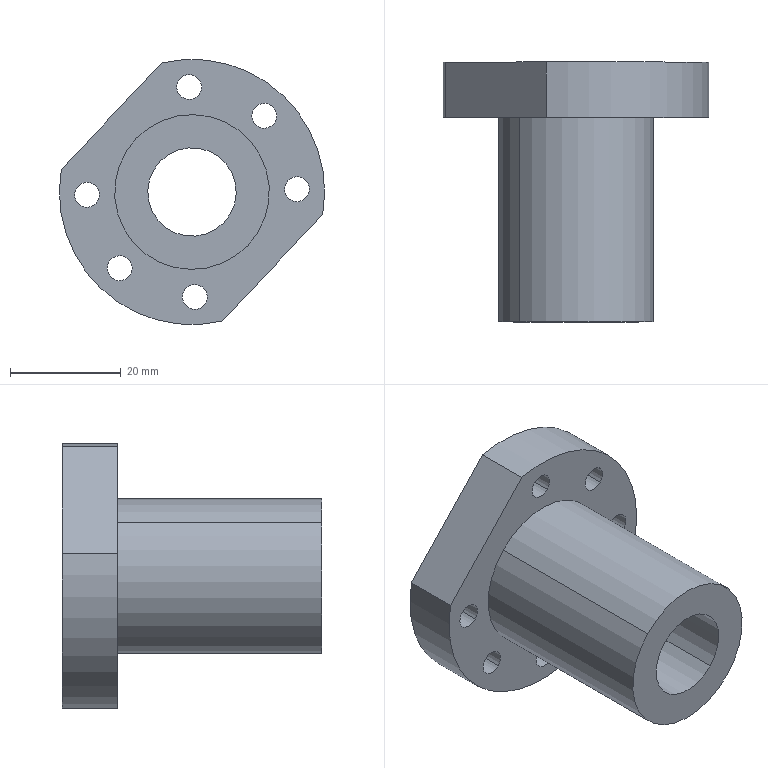Component | SolidWorks | 100-1_Copy(2)-1 | 1 solid | 23 faces | box 48 x 47 x 48 mm | volume 29034 mm3 | cylinder 18 | plane 5 | commonest cylinder face diameters 4.5 x12 16 x2 28 x2 48 x2
STEP:
#1=COLOUR_RGB('',0.7922,0.8196,0.9333);
#2=FILL_AREA_STYLE_COLOUR('',#1);
#3=FILL_AREA_STYLE('',(#2));
#4=SURFACE_STYLE_FILL_AREA(#3);
#5=SURFACE_SIDE_STYLE('',(#4));
#6=SURFACE_STYLE_USAGE(.BOTH.,#5);
#7=PRESENTATION_STYLE_ASSIGNMENT((#6));
#8=CARTESIAN_POINT('',(19.805,43.68,-79.282));
#9=VERTEX_POINT('',#8);
#10=CARTESIAN_POINT('',(19.805,45.53,-79.282));
#11=VERTEX_POINT('',#10);
#12=CARTESIAN_POINT('',(19.805,43.68,-79.282));
#13=DIRECTION('',(-0.,1.,0.));
#14=VECTOR('',#13,39.37);
#15=LINE('',#12,#14);
#16=EDGE_CURVE('',#9,#11,#15,.T.);
#17=ORIENTED_EDGE('',*,*,#16,.F.);
#18=CARTESIAN_POINT('',(19.348,43.68,-78.848));
#19=VERTEX_POINT('',#18);
#20=CARTESIAN_POINT('',(19.576,43.68,-79.065));
#21=DIRECTION('',(-0.,1.,0.));
#22=DIRECTION('',(-0.7258,0.,0.6879));
#23=AXIS2_PLACEMENT_3D('',#20,#21,#22);
#24=CIRCLE('',#23,0.315);
#25=EDGE_CURVE('',#19,#9,#24,.T.);
#26=ORIENTED_EDGE('',*,*,#25,.F.);
#27=CARTESIAN_POINT('',(19.348,45.53,-78.848));
#28=VERTEX_POINT('',#27);
#29=CARTESIAN_POINT('',(19.348,43.68,-78.848));
#30=DIRECTION('',(-0.,1.,0.));
#31=VECTOR('',#30,39.37);
#32=LINE('',#29,#31);
#33=EDGE_CURVE('',#19,#28,#32,.T.);
#34=ORIENTED_EDGE('',*,*,#33,.T.);
#35=CARTESIAN_POINT('',(19.576,45.53,-79.065));
#36=DIRECTION('',(-0.,1.,0.));
#37=DIRECTION('',(-0.7258,0.,0.6879));
#38=AXIS2_PLACEMENT_3D('',#35,#36,#37);
#39=CIRCLE('',#38,0.315);
#40=EDGE_CURVE('',#28,#11,#39,.T.);
#41=ORIENTED_EDGE('',*,*,#40,.T.);
#42=EDGE_LOOP('',(#17,#26,#34,#41));
#43=FACE_OUTER_BOUND('',#42,.T.);
#44=CARTESIAN_POINT('',(19.576,43.68,-79.065));
#45=DIRECTION('',(-0.,1.,0.));
#46=DIRECTION('',(-0.7258,0.,0.6879));
#47=AXIS2_PLACEMENT_3D('',#44,#45,#46);
#48=CYLINDRICAL_SURFACE('',#47,0.315);
#49=ADVANCED_FACE('',(#43),#48,.F.);
#50=ORIENTED_EDGE('',*,*,#25,.T.);
#51=CARTESIAN_POINT('',(19.576,43.68,-79.065));
#52=DIRECTION('',(-0.,1.,0.));
#53=DIRECTION('',(-0.7258,0.,0.6879));
#54=AXIS2_PLACEMENT_3D('',#51,#52,#53);
#55=CIRCLE('',#54,0.315);
#56=EDGE_CURVE('',#9,#19,#55,.T.);
#57=ORIENTED_EDGE('',*,*,#56,.T.);
#58=EDGE_LOOP('',(#50,#57));
#59=FACE_BOUND('',#58,.T.);
#60=CARTESIAN_POINT('',(19.176,43.68,-78.686));
#61=VERTEX_POINT('',#60);
#62=CARTESIAN_POINT('',(19.976,43.68,-79.444));
#63=VERTEX_POINT('',#62);
#64=CARTESIAN_POINT('',(19.576,43.68,-79.065));
#65=DIRECTION('',(0.,-1.,-0.));
#66=DIRECTION('',(0.7258,0.,-0.6879));
#67=AXIS2_PLACEMENT_3D('',#64,#65,#66);
#68=CIRCLE('',#67,0.5512);
#69=EDGE_CURVE('',#61,#63,#68,.T.);
#70=ORIENTED_EDGE('',*,*,#69,.T.);
#71=CARTESIAN_POINT('',(19.576,43.68,-79.065));
#72=DIRECTION('',(0.,-1.,-0.));
#73=DIRECTION('',(0.7258,0.,-0.6879));
#74=AXIS2_PLACEMENT_3D('',#71,#72,#73);
#75=CIRCLE('',#74,0.5512);
#76=EDGE_CURVE('',#63,#61,#75,.T.);
#77=ORIENTED_EDGE('',*,*,#76,.T.);
#78=EDGE_LOOP('',(#70,#77));
#79=FACE_OUTER_BOUND('',#78,.T.);
#80=CARTESIAN_POINT('',(19.576,43.68,-79.065));
#81=DIRECTION('',(0.,-1.,-0.));
#82=DIRECTION('',(0.7258,0.,-0.6879));
#83=AXIS2_PLACEMENT_3D('',#80,#81,#82);
#84=PLANE('',#83);
#85=ADVANCED_FACE('',(#59,#79),#84,.T.);
#86=CARTESIAN_POINT('',(19.976,45.136,-79.444));
#87=VERTEX_POINT('',#86);
#88=CARTESIAN_POINT('',(19.976,43.68,-79.444));
#89=DIRECTION('',(-0.,1.,0.));
#90=VECTOR('',#89,39.37);
#91=LINE('',#88,#90);
#92=EDGE_CURVE('',#63,#87,#91,.T.);
#93=ORIENTED_EDGE('',*,*,#92,.F.);
#94=ORIENTED_EDGE('',*,*,#69,.F.);
#95=CARTESIAN_POINT('',(19.176,45.136,-78.686));
#96=VERTEX_POINT('',#95);
#97=CARTESIAN_POINT('',(19.176,43.68,-78.686));
#98=DIRECTION('',(-0.,1.,0.));
#99=VECTOR('',#98,39.37);
#100=LINE('',#97,#99);
#101=EDGE_CURVE('',#61,#96,#100,.T.);
#102=ORIENTED_EDGE('',*,*,#101,.T.);
#103=CARTESIAN_POINT('',(19.576,45.136,-79.065));
#104=DIRECTION('',(0.,-1.,-0.));
#105=DIRECTION('',(-0.7258,0.,0.6879));
#106=AXIS2_PLACEMENT_3D('',#103,#104,#105);
#107=CIRCLE('',#106,0.5512);
#108=EDGE_CURVE('',#96,#87,#107,.T.);
#109=ORIENTED_EDGE('',*,*,#108,.T.);
#110=EDGE_LOOP('',(#93,#94,#102,#109));
#111=FACE_OUTER_BOUND('',#110,.T.);
#112=CARTESIAN_POINT('',(19.576,43.68,-79.065));
#113=DIRECTION('',(-0.,1.,0.));
#114=DIRECTION('',(-0.7258,0.,0.6879));
#115=AXIS2_PLACEMENT_3D('',#112,#113,#114);
#116=CYLINDRICAL_SURFACE('',#115,0.5512);
#117=ADVANCED_FACE('',(#111),#116,.T.);
#118=CARTESIAN_POINT('',(20.026,45.53,-78.461));
#119=VERTEX_POINT('',#118);
#120=CARTESIAN_POINT('',(20.026,45.136,-78.461));
#121=VERTEX_POINT('',#120);
#122=CARTESIAN_POINT('',(20.026,45.136,-78.461));
#123=DIRECTION('',(0.,-1.,-0.));
#124=VECTOR('',#123,39.37);
#125=LINE('',#122,#124);
#126=EDGE_CURVE('',#119,#121,#125,.T.);
#127=ORIENTED_EDGE('',*,*,#126,.F.);
#128=CARTESIAN_POINT('',(20.155,45.53,-78.583));
#129=VERTEX_POINT('',#128);
#130=CARTESIAN_POINT('',(20.091,45.53,-78.522));
#131=DIRECTION('',(0.,-1.,-0.));
#132=DIRECTION('',(0.7258,0.,-0.6879));
#133=AXIS2_PLACEMENT_3D('',#130,#131,#132);
#134=CIRCLE('',#133,0.08858);
#135=EDGE_CURVE('',#129,#119,#134,.T.);
#136=ORIENTED_EDGE('',*,*,#135,.F.);
#137=CARTESIAN_POINT('',(20.155,45.136,-78.583));
#138=VERTEX_POINT('',#137);
#139=CARTESIAN_POINT('',(20.155,45.136,-78.583));
#140=DIRECTION('',(0.,-1.,-0.));
#141=VECTOR('',#140,39.37);
#142=LINE('',#139,#141);
#143=EDGE_CURVE('',#129,#138,#142,.T.);
#144=ORIENTED_EDGE('',*,*,#143,.T.);
#145=CARTESIAN_POINT('',(20.091,45.136,-78.522));
#146=DIRECTION('',(0.,-1.,-0.));
#147=DIRECTION('',(0.7258,0.,-0.6879));
#148=AXIS2_PLACEMENT_3D('',#145,#146,#147);
#149=CIRCLE('',#148,0.08858);
#150=EDGE_CURVE('',#138,#121,#149,.T.);
#151=ORIENTED_EDGE('',*,*,#150,.T.);
#152=EDGE_LOOP('',(#127,#136,#144,#151));
#153=FACE_OUTER_BOUND('',#152,.T.);
#154=CARTESIAN_POINT('',(20.091,45.136,-78.522));
#155=DIRECTION('',(0.,-1.,-0.));
#156=DIRECTION('',(0.7258,0.,-0.6879));
#157=AXIS2_PLACEMENT_3D('',#154,#155,#156);
#158=CYLINDRICAL_SURFACE('',#157,0.08858);
#159=ADVANCED_FACE('',(#153),#158,.F.);
#160=CARTESIAN_POINT('',(19.492,45.53,-78.256));
#161=VERTEX_POINT('',#160);
#162=CARTESIAN_POINT('',(19.492,45.136,-78.256));
#163=VERTEX_POINT('',#162);
#164=CARTESIAN_POINT('',(19.492,45.136,-78.256));
#165=DIRECTION('',(0.,-1.,-0.));
#166=VECTOR('',#165,39.37);
#167=LINE('',#164,#166);
#168=EDGE_CURVE('',#161,#163,#167,.T.);
#169=ORIENTED_EDGE('',*,*,#168,.F.);
#170=CARTESIAN_POINT('',(19.62,45.53,-78.378));
#171=VERTEX_POINT('',#170);
#172=CARTESIAN_POINT('',(19.556,45.53,-78.317));
#173=DIRECTION('',(0.,-1.,-0.));
#174=DIRECTION('',(0.7258,0.,-0.6879));
#175=AXIS2_PLACEMENT_3D('',#172,#173,#174);
#176=CIRCLE('',#175,0.08858);
#177=EDGE_CURVE('',#171,#161,#176,.T.);
#178=ORIENTED_EDGE('',*,*,#177,.F.);
#179=CARTESIAN_POINT('',(19.62,45.136,-78.378));
#180=VERTEX_POINT('',#179);
#181=CARTESIAN_POINT('',(19.62,45.136,-78.378));
#182=DIRECTION('',(0.,-1.,-0.));
#183=VECTOR('',#182,39.37);
#184=LINE('',#181,#183);
#185=EDGE_CURVE('',#171,#180,#184,.T.);
#186=ORIENTED_EDGE('',*,*,#185,.T.);
#187=CARTESIAN_POINT('',(19.556,45.136,-78.317));
#188=DIRECTION('',(0.,-1.,-0.));
#189=DIRECTION('',(0.7258,0.,-0.6879));
#190=AXIS2_PLACEMENT_3D('',#187,#188,#189);
#191=CIRCLE('',#190,0.08858);
#192=EDGE_CURVE('',#180,#163,#191,.T.);
#193=ORIENTED_EDGE('',*,*,#192,.T.);
#194=EDGE_LOOP('',(#169,#178,#186,#193));
#195=FACE_OUTER_BOUND('',#194,.T.);
#196=CARTESIAN_POINT('',(19.556,45.136,-78.317));
#197=DIRECTION('',(0.,-1.,-0.));
#198=DIRECTION('',(0.7258,0.,-0.6879));
#199=AXIS2_PLACEMENT_3D('',#196,#197,#198);
#200=CYLINDRICAL_SURFACE('',#199,0.08858);
#201=ADVANCED_FACE('',(#195),#200,.F.);
#202=CARTESIAN_POINT('',(18.764,45.53,-79.024));
#203=VERTEX_POINT('',#202);
#204=CARTESIAN_POINT('',(18.764,45.136,-79.024));
#205=VERTEX_POINT('',#204);
#206=CARTESIAN_POINT('',(18.764,45.136,-79.024));
#207=DIRECTION('',(0.,-1.,-0.));
#208=VECTOR('',#207,39.37);
#209=LINE('',#206,#208);
#210=EDGE_CURVE('',#203,#205,#209,.T.);
#211=ORIENTED_EDGE('',*,*,#210,.F.);
#212=CARTESIAN_POINT('',(18.893,45.53,-79.146));
#213=VERTEX_POINT('',#212);
#214=CARTESIAN_POINT('',(18.828,45.53,-79.085));
#215=DIRECTION('',(0.,-1.,-0.));
#216=DIRECTION('',(0.7258,0.,-0.6879));
#217=AXIS2_PLACEMENT_3D('',#214,#215,#216);
#218=CIRCLE('',#217,0.08858);
#219=EDGE_CURVE('',#213,#203,#218,.T.);
#220=ORIENTED_EDGE('',*,*,#219,.F.);
#221=CARTESIAN_POINT('',(18.893,45.136,-79.146));
#222=VERTEX_POINT('',#221);
#223=CARTESIAN_POINT('',(18.893,45.136,-79.146));
#224=DIRECTION('',(0.,-1.,-0.));
#225=VECTOR('',#224,39.37);
#226=LINE('',#223,#225);
#227=EDGE_CURVE('',#213,#222,#226,.T.);
#228=ORIENTED_EDGE('',*,*,#227,.T.);
#229=CARTESIAN_POINT('',(18.828,45.136,-79.085));
#230=DIRECTION('',(0.,-1.,-0.));
#231=DIRECTION('',(0.7258,0.,-0.6879));
#232=AXIS2_PLACEMENT_3D('',#229,#230,#231);
#233=CIRCLE('',#232,0.08858);
#234=EDGE_CURVE('',#222,#205,#233,.T.);
#235=ORIENTED_EDGE('',*,*,#234,.T.);
#236=EDGE_LOOP('',(#211,#220,#228,#235));
#237=FACE_OUTER_BOUND('',#236,.T.);
#238=CARTESIAN_POINT('',(18.828,45.136,-79.085));
#239=DIRECTION('',(0.,-1.,-0.));
#240=DIRECTION('',(0.7258,0.,-0.6879));
#241=AXIS2_PLACEMENT_3D('',#238,#239,#240);
#242=CYLINDRICAL_SURFACE('',#241,0.08858);
#243=ADVANCED_FACE('',(#237),#242,.F.);
#244=CARTESIAN_POINT('',(19.532,45.53,-79.752));
#245=VERTEX_POINT('',#244);
#246=CARTESIAN_POINT('',(19.532,45.136,-79.752));
#247=VERTEX_POINT('',#246);
#248=CARTESIAN_POINT('',(19.532,45.136,-79.752));
#249=DIRECTION('',(0.,-1.,-0.));
#250=VECTOR('',#249,39.37);
#251=LINE('',#248,#250);
#252=EDGE_CURVE('',#245,#247,#251,.T.);
#253=ORIENTED_EDGE('',*,*,#252,.F.);
#254=CARTESIAN_POINT('',(19.66,45.53,-79.874));
#255=VERTEX_POINT('',#254);
#256=CARTESIAN_POINT('',(19.596,45.53,-79.813));
#257=DIRECTION('',(0.,-1.,-0.));
#258=DIRECTION('',(0.7258,0.,-0.6879));
#259=AXIS2_PLACEMENT_3D('',#256,#257,#258);
#260=CIRCLE('',#259,0.08858);
#261=EDGE_CURVE('',#255,#245,#260,.T.);
#262=ORIENTED_EDGE('',*,*,#261,.F.);
#263=CARTESIAN_POINT('',(19.66,45.136,-79.874));
#264=VERTEX_POINT('',#263);
#265=CARTESIAN_POINT('',(19.66,45.136,-79.874));
#266=DIRECTION('',(0.,-1.,-0.));
#267=VECTOR('',#266,39.37);
#268=LINE('',#265,#267);
#269=EDGE_CURVE('',#255,#264,#268,.T.);
#270=ORIENTED_EDGE('',*,*,#269,.T.);
#271=CARTESIAN_POINT('',(19.596,45.136,-79.813));
#272=DIRECTION('',(0.,-1.,-0.));
#273=DIRECTION('',(0.7258,0.,-0.6879));
#274=AXIS2_PLACEMENT_3D('',#271,#272,#273);
#275=CIRCLE('',#274,0.08858);
#276=EDGE_CURVE('',#264,#247,#275,.T.);
#277=ORIENTED_EDGE('',*,*,#276,.T.);
#278=EDGE_LOOP('',(#253,#262,#270,#277));
#279=FACE_OUTER_BOUND('',#278,.T.);
#280=CARTESIAN_POINT('',(19.596,45.136,-79.813));
#281=DIRECTION('',(0.,-1.,-0.));
#282=DIRECTION('',(0.7258,0.,-0.6879));
#283=AXIS2_PLACEMENT_3D('',#280,#281,#282);
#284=CYLINDRICAL_SURFACE('',#283,0.08858);
#285=ADVANCED_FACE('',(#279),#284,.F.);
#286=CARTESIAN_POINT('',(18.997,45.53,-79.547));
#287=VERTEX_POINT('',#286);
#288=CARTESIAN_POINT('',(18.997,45.136,-79.547));
#289=VERTEX_POINT('',#288);
#290=CARTESIAN_POINT('',(18.997,45.136,-79.547));
#291=DIRECTION('',(0.,-1.,-0.));
#292=VECTOR('',#291,39.37);
#293=LINE('',#290,#292);
#294=EDGE_CURVE('',#287,#289,#293,.T.);
#295=ORIENTED_EDGE('',*,*,#294,.F.);
#296=CARTESIAN_POINT('',(19.126,45.53,-79.669));
#297=VERTEX_POINT('',#296);
#298=CARTESIAN_POINT('',(19.062,45.53,-79.608));
#299=DIRECTION('',(0.,-1.,-0.));
#300=DIRECTION('',(0.7258,0.,-0.6879));
#301=AXIS2_PLACEMENT_3D('',#298,#299,#300);
#302=CIRCLE('',#301,0.08858);
#303=EDGE_CURVE('',#297,#287,#302,.T.);
#304=ORIENTED_EDGE('',*,*,#303,.F.);
#305=CARTESIAN_POINT('',(19.126,45.136,-79.669));
#306=VERTEX_POINT('',#305);
#307=CARTESIAN_POINT('',(19.126,45.136,-79.669));
#308=DIRECTION('',(0.,-1.,-0.));
#309=VECTOR('',#308,39.37);
#310=LINE('',#307,#309);
#311=EDGE_CURVE('',#297,#306,#310,.T.);
#312=ORIENTED_EDGE('',*,*,#311,.T.);
#313=CARTESIAN_POINT('',(19.062,45.136,-79.608));
#314=DIRECTION('',(0.,-1.,-0.));
#315=DIRECTION('',(0.7258,0.,-0.6879));
#316=AXIS2_PLACEMENT_3D('',#313,#314,#315);
#317=CIRCLE('',#316,0.08858);
#318=EDGE_CURVE('',#306,#289,#317,.T.);
#319=ORIENTED_EDGE('',*,*,#318,.T.);
#320=EDGE_LOOP('',(#295,#304,#312,#319));
#321=FACE_OUTER_BOUND('',#320,.T.);
#322=CARTESIAN_POINT('',(19.062,45.136,-79.608));
#323=DIRECTION('',(0.,-1.,-0.));
#324=DIRECTION('',(0.7258,0.,-0.6879));
#325=AXIS2_PLACEMENT_3D('',#322,#323,#324);
#326=CYLINDRICAL_SURFACE('',#325,0.08858);
#327=ADVANCED_FACE('',(#321),#326,.F.);
#328=CARTESIAN_POINT('',(20.26,45.53,-78.984));
#329=VERTEX_POINT('',#328);
#330=CARTESIAN_POINT('',(20.26,45.136,-78.984));
#331=VERTEX_POINT('',#330);
#332=CARTESIAN_POINT('',(20.26,45.136,-78.984));
#333=DIRECTION('',(0.,-1.,-0.));
#334=VECTOR('',#333,39.37);
#335=LINE('',#332,#334);
#336=EDGE_CURVE('',#329,#331,#335,.T.);
#337=ORIENTED_EDGE('',*,*,#336,.F.);
#338=CARTESIAN_POINT('',(20.388,45.53,-79.106));
#339=VERTEX_POINT('',#338);
#340=CARTESIAN_POINT('',(20.324,45.53,-79.045));
#341=DIRECTION('',(0.,-1.,-0.));
#342=DIRECTION('',(0.7258,0.,-0.6879));
#343=AXIS2_PLACEMENT_3D('',#340,#341,#342);
#344=CIRCLE('',#343,0.08858);
#345=EDGE_CURVE('',#339,#329,#344,.T.);
#346=ORIENTED_EDGE('',*,*,#345,.F.);
#347=CARTESIAN_POINT('',(20.388,45.136,-79.106));
#348=VERTEX_POINT('',#347);
#349=CARTESIAN_POINT('',(20.388,45.136,-79.106));
#350=DIRECTION('',(0.,-1.,-0.));
#351=VECTOR('',#350,39.37);
#352=LINE('',#349,#351);
#353=EDGE_CURVE('',#339,#348,#352,.T.);
#354=ORIENTED_EDGE('',*,*,#353,.T.);
#355=CARTESIAN_POINT('',(20.324,45.136,-79.045));
#356=DIRECTION('',(0.,-1.,-0.));
#357=DIRECTION('',(0.7258,0.,-0.6879));
#358=AXIS2_PLACEMENT_3D('',#355,#356,#357);
#359=CIRCLE('',#358,0.08858);
#360=EDGE_CURVE('',#348,#331,#359,.T.);
#361=ORIENTED_EDGE('',*,*,#360,.T.);
#362=EDGE_LOOP('',(#337,#346,#354,#361));
#363=FACE_OUTER_BOUND('',#362,.T.);
#364=CARTESIAN_POINT('',(20.324,45.136,-79.045));
#365=DIRECTION('',(0.,-1.,-0.));
#366=DIRECTION('',(0.7258,0.,-0.6879));
#367=AXIS2_PLACEMENT_3D('',#364,#365,#366);
#368=CYLINDRICAL_SURFACE('',#367,0.08858);
#369=ADVANCED_FACE('',(#363),#368,.F.);
#370=ORIENTED_EDGE('',*,*,#345,.T.);
#371=CARTESIAN_POINT('',(20.324,45.53,-79.045));
#372=DIRECTION('',(0.,-1.,-0.));
#373=DIRECTION('',(0.7258,0.,-0.6879));
#374=AXIS2_PLACEMENT_3D('',#371,#372,#373);
#375=CIRCLE('',#374,0.08858);
#376=EDGE_CURVE('',#329,#339,#375,.T.);
#377=ORIENTED_EDGE('',*,*,#376,.T.);
#378=EDGE_LOOP('',(#370,#377));
#379=FACE_BOUND('',#378,.T.);
#380=ORIENTED_EDGE('',*,*,#303,.T.);
#381=CARTESIAN_POINT('',(19.062,45.53,-79.608));
#382=DIRECTION('',(0.,-1.,-0.));
#383=DIRECTION('',(0.7258,0.,-0.6879));
#384=AXIS2_PLACEMENT_3D('',#381,#382,#383);
#385=CIRCLE('',#384,0.08858);
#386=EDGE_CURVE('',#287,#297,#385,.T.);
#387=ORIENTED_EDGE('',*,*,#386,.T.);
#388=EDGE_LOOP('',(#380,#387));
#389=FACE_BOUND('',#388,.T.);
#390=ORIENTED_EDGE('',*,*,#261,.T.);
#391=CARTESIAN_POINT('',(19.596,45.53,-79.813));
#392=DIRECTION('',(0.,-1.,-0.));
#393=DIRECTION('',(0.7258,0.,-0.6879));
#394=AXIS2_PLACEMENT_3D('',#391,#392,#393);
#395=CIRCLE('',#394,0.08858);
#396=EDGE_CURVE('',#245,#255,#395,.T.);
#397=ORIENTED_EDGE('',*,*,#396,.T.);
#398=EDGE_LOOP('',(#390,#397));
#399=FACE_BOUND('',#398,.T.);
#400=ORIENTED_EDGE('',*,*,#219,.T.);
#401=CARTESIAN_POINT('',(18.828,45.53,-79.085));
#402=DIRECTION('',(0.,-1.,-0.));
#403=DIRECTION('',(0.7258,0.,-0.6879));
#404=AXIS2_PLACEMENT_3D('',#401,#402,#403);
#405=CIRCLE('',#404,0.08858);
#406=EDGE_CURVE('',#203,#213,#405,.T.);
#407=ORIENTED_EDGE('',*,*,#406,.T.);
#408=EDGE_LOOP('',(#400,#407));
#409=FACE_BOUND('',#408,.T.);
#410=ORIENTED_EDGE('',*,*,#177,.T.);
#411=CARTESIAN_POINT('',(19.556,45.53,-78.317));
#412=DIRECTION('',(0.,-1.,-0.));
#413=DIRECTION('',(0.7258,0.,-0.6879));
#414=AXIS2_PLACEMENT_3D('',#411,#412,#413);
#415=CIRCLE('',#414,0.08858);
#416=EDGE_CURVE('',#161,#171,#415,.T.);
#417=ORIENTED_EDGE('',*,*,#416,.T.);
#418=EDGE_LOOP('',(#410,#417));
#419=FACE_BOUND('',#418,.T.);
#420=ORIENTED_EDGE('',*,*,#135,.T.);
#421=CARTESIAN_POINT('',(20.091,45.53,-78.522));
#422=DIRECTION('',(0.,-1.,-0.));
#423=DIRECTION('',(0.7258,0.,-0.6879));
#424=AXIS2_PLACEMENT_3D('',#421,#422,#423);
#425=CIRCLE('',#424,0.08858);
#426=EDGE_CURVE('',#119,#129,#425,.T.);
#427=ORIENTED_EDGE('',*,*,#426,.T.);
#428=EDGE_LOOP('',(#420,#427));
#429=FACE_BOUND('',#428,.T.);
#430=ORIENTED_EDGE('',*,*,#40,.F.);
#431=CARTESIAN_POINT('',(19.576,45.53,-79.065));
#432=DIRECTION('',(-0.,1.,0.));
#433=DIRECTION('',(-0.7258,0.,0.6879));
#434=AXIS2_PLACEMENT_3D('',#431,#432,#433);
#435=CIRCLE('',#434,0.315);
#436=EDGE_CURVE('',#11,#28,#435,.T.);
#437=ORIENTED_EDGE('',*,*,#436,.F.);
#438=EDGE_LOOP('',(#430,#437));
#439=FACE_BOUND('',#438,.T.);
#440=CARTESIAN_POINT('',(19.364,45.53,-78.144));
#441=VERTEX_POINT('',#440);
#442=CARTESIAN_POINT('',(20.507,45.53,-79.227));
#443=VERTEX_POINT('',#442);
#444=CARTESIAN_POINT('',(19.576,45.53,-79.065));
#445=DIRECTION('',(-0.,1.,0.));
#446=DIRECTION('',(-0.7258,0.,0.6879));
#447=AXIS2_PLACEMENT_3D('',#444,#445,#446);
#448=CIRCLE('',#447,0.9449);
#449=EDGE_CURVE('',#441,#443,#448,.T.);
#450=ORIENTED_EDGE('',*,*,#449,.T.);
#451=CARTESIAN_POINT('',(19.788,45.53,-79.986));
#452=VERTEX_POINT('',#451);
#453=CARTESIAN_POINT('',(20.507,45.53,-79.227));
#454=DIRECTION('',(-0.6879,-0.,-0.7258));
#455=VECTOR('',#454,39.37);
#456=LINE('',#453,#455);
#457=EDGE_CURVE('',#443,#452,#456,.T.);
#458=ORIENTED_EDGE('',*,*,#457,.T.);
#459=CARTESIAN_POINT('',(18.645,45.53,-78.902));
#460=VERTEX_POINT('',#459);
#461=CARTESIAN_POINT('',(19.576,45.53,-79.065));
#462=DIRECTION('',(-0.,1.,0.));
#463=DIRECTION('',(-0.7258,0.,0.6879));
#464=AXIS2_PLACEMENT_3D('',#461,#462,#463);
#465=CIRCLE('',#464,0.9449);
#466=EDGE_CURVE('',#452,#460,#465,.T.);
#467=ORIENTED_EDGE('',*,*,#466,.T.);
#468=CARTESIAN_POINT('',(18.645,45.53,-78.902));
#469=DIRECTION('',(0.6879,0.,0.7258));
#470=VECTOR('',#469,39.37);
#471=LINE('',#468,#470);
#472=EDGE_CURVE('',#460,#441,#471,.T.);
#473=ORIENTED_EDGE('',*,*,#472,.T.);
#474=EDGE_LOOP('',(#450,#458,#467,#473));
#475=FACE_OUTER_BOUND('',#474,.T.);
#476=CARTESIAN_POINT('',(19.576,45.53,-79.065));
#477=DIRECTION('',(-0.,1.,0.));
#478=DIRECTION('',(0.6879,0.,0.7258));
#479=AXIS2_PLACEMENT_3D('',#476,#477,#478);
#480=PLANE('',#479);
#481=ADVANCED_FACE('',(#379,#389,#399,#409,#419,#429,#439,#475),#480,.T.);
#482=CARTESIAN_POINT('',(18.645,45.136,-78.902));
#483=VERTEX_POINT('',#482);
#484=CARTESIAN_POINT('',(19.364,45.136,-78.144));
#485=VERTEX_POINT('',#484);
#486=CARTESIAN_POINT('',(18.645,45.136,-78.902));
#487=DIRECTION('',(0.6879,0.,0.7258));
#488=VECTOR('',#487,39.37);
#489=LINE('',#486,#488);
#490=EDGE_CURVE('',#483,#485,#489,.T.);
#491=ORIENTED_EDGE('',*,*,#490,.T.);
#492=CARTESIAN_POINT('',(19.364,45.53,-78.144));
#493=DIRECTION('',(0.,-1.,-0.));
#494=VECTOR('',#493,39.37);
#495=LINE('',#492,#494);
#496=EDGE_CURVE('',#441,#485,#495,.T.);
#497=ORIENTED_EDGE('',*,*,#496,.F.);
#498=ORIENTED_EDGE('',*,*,#472,.F.);
#499=CARTESIAN_POINT('',(18.645,45.53,-78.902));
#500=DIRECTION('',(0.,-1.,-0.));
#501=VECTOR('',#500,39.37);
#502=LINE('',#499,#501);
#503=EDGE_CURVE('',#460,#483,#502,.T.);
#504=ORIENTED_EDGE('',*,*,#503,.T.);
#505=EDGE_LOOP('',(#491,#497,#498,#504));
#506=FACE_OUTER_BOUND('',#505,.T.);
#507=CARTESIAN_POINT('',(18.645,45.53,-78.902));
#508=DIRECTION('',(0.7258,0.,-0.6879));
#509=DIRECTION('',(-0.6879,-0.,-0.7258));
#510=AXIS2_PLACEMENT_3D('',#507,#508,#509);
#511=PLANE('',#510);
#512=ADVANCED_FACE('',(#506),#511,.F.);
#513=CARTESIAN_POINT('',(19.788,45.136,-79.986));
#514=VERTEX_POINT('',#513);
#515=CARTESIAN_POINT('',(19.576,45.136,-79.065));
#516=DIRECTION('',(-0.,1.,0.));
#517=DIRECTION('',(-0.7258,0.,0.6879));
#518=AXIS2_PLACEMENT_3D('',#515,#516,#517);
#519=CIRCLE('',#518,0.9449);
#520=EDGE_CURVE('',#514,#483,#519,.T.);
#521=ORIENTED_EDGE('',*,*,#520,.T.);
#522=ORIENTED_EDGE('',*,*,#503,.F.);
#523=ORIENTED_EDGE('',*,*,#466,.F.);
#524=CARTESIAN_POINT('',(19.788,45.53,-79.986));
#525=DIRECTION('',(0.,-1.,-0.));
#526=VECTOR('',#525,39.37);
#527=LINE('',#524,#526);
#528=EDGE_CURVE('',#452,#514,#527,.T.);
#529=ORIENTED_EDGE('',*,*,#528,.T.);
#530=EDGE_LOOP('',(#521,#522,#523,#529));
#531=FACE_OUTER_BOUND('',#530,.T.);
#532=CARTESIAN_POINT('',(19.576,45.53,-79.065));
#533=DIRECTION('',(0.,-1.,-0.));
#534=DIRECTION('',(0.7258,0.,-0.6879));
#535=AXIS2_PLACEMENT_3D('',#532,#533,#534);
#536=CYLINDRICAL_SURFACE('',#535,0.9449);
#537=ADVANCED_FACE('',(#531),#536,.T.);
#538=CARTESIAN_POINT('',(20.507,45.136,-79.227));
#539=VERTEX_POINT('',#538);
#540=CARTESIAN_POINT('',(20.507,45.136,-79.227));
#541=DIRECTION('',(-0.6879,-0.,-0.7258));
#542=VECTOR('',#541,39.37);
#543=LINE('',#540,#542);
#544=EDGE_CURVE('',#539,#514,#543,.T.);
#545=ORIENTED_EDGE('',*,*,#544,.T.);
#546=ORIENTED_EDGE('',*,*,#528,.F.);
#547=ORIENTED_EDGE('',*,*,#457,.F.);
#548=CARTESIAN_POINT('',(20.507,45.53,-79.227));
#549=DIRECTION('',(0.,-1.,-0.));
#550=VECTOR('',#549,39.37);
#551=LINE('',#548,#550);
#552=EDGE_CURVE('',#443,#539,#551,.T.);
#553=ORIENTED_EDGE('',*,*,#552,.T.);
#554=EDGE_LOOP('',(#545,#546,#547,#553));
#555=FACE_OUTER_BOUND('',#554,.T.);
#556=CARTESIAN_POINT('',(20.507,45.53,-79.227));
#557=DIRECTION('',(-0.7258,-0.,0.6879));
#558=DIRECTION('',(0.6879,0.,0.7258));
#559=AXIS2_PLACEMENT_3D('',#556,#557,#558);
#560=PLANE('',#559);
#561=ADVANCED_FACE('',(#555),#560,.F.);
#562=CARTESIAN_POINT('',(19.576,45.136,-79.065));
#563=DIRECTION('',(-0.,1.,0.));
#564=DIRECTION('',(-0.7258,0.,0.6879));
#565=AXIS2_PLACEMENT_3D('',#562,#563,#564);
#566=CIRCLE('',#565,0.9449);
#567=EDGE_CURVE('',#485,#539,#566,.T.);
#568=ORIENTED_EDGE('',*,*,#567,.T.);
#569=ORIENTED_EDGE('',*,*,#552,.F.);
#570=ORIENTED_EDGE('',*,*,#449,.F.);
#571=ORIENTED_EDGE('',*,*,#496,.T.);
#572=EDGE_LOOP('',(#568,#569,#570,#571));
#573=FACE_OUTER_BOUND('',#572,.T.);
#574=CARTESIAN_POINT('',(19.576,45.53,-79.065));
#575=DIRECTION('',(0.,-1.,-0.));
#576=DIRECTION('',(0.7258,0.,-0.6879));
#577=AXIS2_PLACEMENT_3D('',#574,#575,#576);
#578=CYLINDRICAL_SURFACE('',#577,0.9449);
#579=ADVANCED_FACE('',(#573),#578,.T.);
#580=ORIENTED_EDGE('',*,*,#108,.F.);
#581=CARTESIAN_POINT('',(19.576,45.136,-79.065));
#582=DIRECTION('',(0.,-1.,-0.));
#583=DIRECTION('',(-0.7258,0.,0.6879));
#584=AXIS2_PLACEMENT_3D('',#581,#582,#583);
#585=CIRCLE('',#584,0.5512);
#586=EDGE_CURVE('',#87,#96,#585,.T.);
#587=ORIENTED_EDGE('',*,*,#586,.F.);
#588=EDGE_LOOP('',(#580,#587));
#589=FACE_BOUND('',#588,.T.);
#590=ORIENTED_EDGE('',*,*,#360,.F.);
#591=CARTESIAN_POINT('',(20.324,45.136,-79.045));
#592=DIRECTION('',(0.,-1.,-0.));
#593=DIRECTION('',(0.7258,0.,-0.6879));
#594=AXIS2_PLACEMENT_3D('',#591,#592,#593);
#595=CIRCLE('',#594,0.08858);
#596=EDGE_CURVE('',#331,#348,#595,.T.);
#597=ORIENTED_EDGE('',*,*,#596,.F.);
#598=EDGE_LOOP('',(#590,#597));
#599=FACE_BOUND('',#598,.T.);
#600=ORIENTED_EDGE('',*,*,#318,.F.);
#601=CARTESIAN_POINT('',(19.062,45.136,-79.608));
#602=DIRECTION('',(0.,-1.,-0.));
#603=DIRECTION('',(0.7258,0.,-0.6879));
#604=AXIS2_PLACEMENT_3D('',#601,#602,#603);
#605=CIRCLE('',#604,0.08858);
#606=EDGE_CURVE('',#289,#306,#605,.T.);
#607=ORIENTED_EDGE('',*,*,#606,.F.);
#608=EDGE_LOOP('',(#600,#607));
#609=FACE_BOUND('',#608,.T.);
#610=ORIENTED_EDGE('',*,*,#276,.F.);
#611=CARTESIAN_POINT('',(19.596,45.136,-79.813));
#612=DIRECTION('',(0.,-1.,-0.));
#613=DIRECTION('',(0.7258,0.,-0.6879));
#614=AXIS2_PLACEMENT_3D('',#611,#612,#613);
#615=CIRCLE('',#614,0.08858);
#616=EDGE_CURVE('',#247,#264,#615,.T.);
#617=ORIENTED_EDGE('',*,*,#616,.F.);
#618=EDGE_LOOP('',(#610,#617));
#619=FACE_BOUND('',#618,.T.);
#620=ORIENTED_EDGE('',*,*,#234,.F.);
#621=CARTESIAN_POINT('',(18.828,45.136,-79.085));
#622=DIRECTION('',(0.,-1.,-0.));
#623=DIRECTION('',(0.7258,0.,-0.6879));
#624=AXIS2_PLACEMENT_3D('',#621,#622,#623);
#625=CIRCLE('',#624,0.08858);
#626=EDGE_CURVE('',#205,#222,#625,.T.);
#627=ORIENTED_EDGE('',*,*,#626,.F.);
#628=EDGE_LOOP('',(#620,#627));
#629=FACE_BOUND('',#628,.T.);
#630=ORIENTED_EDGE('',*,*,#192,.F.);
#631=CARTESIAN_POINT('',(19.556,45.136,-78.317));
#632=DIRECTION('',(0.,-1.,-0.));
#633=DIRECTION('',(0.7258,0.,-0.6879));
#634=AXIS2_PLACEMENT_3D('',#631,#632,#633);
#635=CIRCLE('',#634,0.08858);
#636=EDGE_CURVE('',#163,#180,#635,.T.);
#637=ORIENTED_EDGE('',*,*,#636,.F.);
#638=EDGE_LOOP('',(#630,#637));
#639=FACE_BOUND('',#638,.T.);
#640=ORIENTED_EDGE('',*,*,#150,.F.);
#641=CARTESIAN_POINT('',(20.091,45.136,-78.522));
#642=DIRECTION('',(0.,-1.,-0.));
#643=DIRECTION('',(0.7258,0.,-0.6879));
#644=AXIS2_PLACEMENT_3D('',#641,#642,#643);
#645=CIRCLE('',#644,0.08858);
#646=EDGE_CURVE('',#121,#138,#645,.T.);
#647=ORIENTED_EDGE('',*,*,#646,.F.);
#648=EDGE_LOOP('',(#640,#647));
#649=FACE_BOUND('',#648,.T.);
#650=ORIENTED_EDGE('',*,*,#567,.F.);
#651=ORIENTED_EDGE('',*,*,#490,.F.);
#652=ORIENTED_EDGE('',*,*,#520,.F.);
#653=ORIENTED_EDGE('',*,*,#544,.F.);
#654=EDGE_LOOP('',(#650,#651,#652,#653));
#655=FACE_OUTER_BOUND('',#654,.T.);
#656=CARTESIAN_POINT('',(19.576,45.136,-79.065));
#657=DIRECTION('',(-0.,1.,0.));
#658=DIRECTION('',(0.6879,0.,0.7258));
#659=AXIS2_PLACEMENT_3D('',#656,#657,#658);
#660=PLANE('',#659);
#661=ADVANCED_FACE('',(#589,#599,#609,#619,#629,#639,#649,#655),#660,.F.);
#662=ORIENTED_EDGE('',*,*,#376,.F.);
#663=ORIENTED_EDGE('',*,*,#336,.T.);
#664=ORIENTED_EDGE('',*,*,#596,.T.);
#665=ORIENTED_EDGE('',*,*,#353,.F.);
#666=EDGE_LOOP('',(#662,#663,#664,#665));
#667=FACE_OUTER_BOUND('',#666,.T.);
#668=CARTESIAN_POINT('',(20.324,45.136,-79.045));
#669=DIRECTION('',(0.,-1.,-0.));
#670=DIRECTION('',(0.7258,0.,-0.6879));
#671=AXIS2_PLACEMENT_3D('',#668,#669,#670);
#672=CYLINDRICAL_SURFACE('',#671,0.08858);
#673=ADVANCED_FACE('',(#667),#672,.F.);
#674=ORIENTED_EDGE('',*,*,#386,.F.);
#675=ORIENTED_EDGE('',*,*,#294,.T.);
#676=ORIENTED_EDGE('',*,*,#606,.T.);
#677=ORIENTED_EDGE('',*,*,#311,.F.);
#678=EDGE_LOOP('',(#674,#675,#676,#677));
#679=FACE_OUTER_BOUND('',#678,.T.);
#680=CARTESIAN_POINT('',(19.062,45.136,-79.608));
#681=DIRECTION('',(0.,-1.,-0.));
#682=DIRECTION('',(0.7258,0.,-0.6879));
#683=AXIS2_PLACEMENT_3D('',#680,#681,#682);
#684=CYLINDRICAL_SURFACE('',#683,0.08858);
#685=ADVANCED_FACE('',(#679),#684,.F.);
#686=ORIENTED_EDGE('',*,*,#396,.F.);
#687=ORIENTED_EDGE('',*,*,#252,.T.);
#688=ORIENTED_EDGE('',*,*,#616,.T.);
#689=ORIENTED_EDGE('',*,*,#269,.F.);
#690=EDGE_LOOP('',(#686,#687,#688,#689));
#691=FACE_OUTER_BOUND('',#690,.T.);
#692=CARTESIAN_POINT('',(19.596,45.136,-79.813));
#693=DIRECTION('',(0.,-1.,-0.));
#694=DIRECTION('',(0.7258,0.,-0.6879));
#695=AXIS2_PLACEMENT_3D('',#692,#693,#694);
#696=CYLINDRICAL_SURFACE('',#695,0.08858);
#697=ADVANCED_FACE('',(#691),#696,.F.);
#698=ORIENTED_EDGE('',*,*,#406,.F.);
#699=ORIENTED_EDGE('',*,*,#210,.T.);
#700=ORIENTED_EDGE('',*,*,#626,.T.);
#701=ORIENTED_EDGE('',*,*,#227,.F.);
#702=EDGE_LOOP('',(#698,#699,#700,#701));
#703=FACE_OUTER_BOUND('',#702,.T.);
#704=CARTESIAN_POINT('',(18.828,45.136,-79.085));
#705=DIRECTION('',(0.,-1.,-0.));
#706=DIRECTION('',(0.7258,0.,-0.6879));
#707=AXIS2_PLACEMENT_3D('',#704,#705,#706);
#708=CYLINDRICAL_SURFACE('',#707,0.08858);
#709=ADVANCED_FACE('',(#703),#708,.F.);
#710=ORIENTED_EDGE('',*,*,#416,.F.);
#711=ORIENTED_EDGE('',*,*,#168,.T.);
#712=ORIENTED_EDGE('',*,*,#636,.T.);
#713=ORIENTED_EDGE('',*,*,#185,.F.);
#714=EDGE_LOOP('',(#710,#711,#712,#713));
#715=FACE_OUTER_BOUND('',#714,.T.);
#716=CARTESIAN_POINT('',(19.556,45.136,-78.317));
#717=DIRECTION('',(0.,-1.,-0.));
#718=DIRECTION('',(0.7258,0.,-0.6879));
#719=AXIS2_PLACEMENT_3D('',#716,#717,#718);
#720=CYLINDRICAL_SURFACE('',#719,0.08858);
#721=ADVANCED_FACE('',(#715),#720,.F.);
#722=ORIENTED_EDGE('',*,*,#426,.F.);
#723=ORIENTED_EDGE('',*,*,#126,.T.);
#724=ORIENTED_EDGE('',*,*,#646,.T.);
#725=ORIENTED_EDGE('',*,*,#143,.F.);
#726=EDGE_LOOP('',(#722,#723,#724,#725));
#727=FACE_OUTER_BOUND('',#726,.T.);
#728=CARTESIAN_POINT('',(20.091,45.136,-78.522));
#729=DIRECTION('',(0.,-1.,-0.));
#730=DIRECTION('',(0.7258,0.,-0.6879));
#731=AXIS2_PLACEMENT_3D('',#728,#729,#730);
#732=CYLINDRICAL_SURFACE('',#731,0.08858);
#733=ADVANCED_FACE('',(#727),#732,.F.);
#734=ORIENTED_EDGE('',*,*,#76,.F.);
#735=ORIENTED_EDGE('',*,*,#92,.T.);
#736=ORIENTED_EDGE('',*,*,#586,.T.);
#737=ORIENTED_EDGE('',*,*,#101,.F.);
#738=EDGE_LOOP('',(#734,#735,#736,#737));
#739=FACE_OUTER_BOUND('',#738,.T.);
#740=CARTESIAN_POINT('',(19.576,43.68,-79.065));
#741=DIRECTION('',(-0.,1.,0.));
#742=DIRECTION('',(-0.7258,0.,0.6879));
#743=AXIS2_PLACEMENT_3D('',#740,#741,#742);
#744=CYLINDRICAL_SURFACE('',#743,0.5512);
#745=ADVANCED_FACE('',(#739),#744,.T.);
#746=ORIENTED_EDGE('',*,*,#56,.F.);
#747=ORIENTED_EDGE('',*,*,#16,.T.);
#748=ORIENTED_EDGE('',*,*,#436,.T.);
#749=ORIENTED_EDGE('',*,*,#33,.F.);
#750=EDGE_LOOP('',(#746,#747,#748,#749));
#751=FACE_OUTER_BOUND('',#750,.T.);
#752=CARTESIAN_POINT('',(19.576,43.68,-79.065));
#753=DIRECTION('',(-0.,1.,0.));
#754=DIRECTION('',(-0.7258,0.,0.6879));
#755=AXIS2_PLACEMENT_3D('',#752,#753,#754);
#756=CYLINDRICAL_SURFACE('',#755,0.315);
#757=ADVANCED_FACE('',(#751),#756,.F.);
#758=CLOSED_SHELL('',(#49,#85,#117,#159,#201,#243,#285,#327,#369,#481,#512,#537,#561,#579,#661,#673,#685,#697,#709,#721,#733,#745,#757));
#759=MANIFOLD_SOLID_BREP('',#758);
#760=STYLED_ITEM('',(#7),#759);
#761=(LENGTH_UNIT()NAMED_UNIT(*)SI_UNIT($,.METRE.));
#762=LENGTH_MEASURE_WITH_UNIT(LENGTH_MEASURE(0.0254),#761);
#763=DIMENSIONAL_EXPONENTS(1.,0.,0.,0.,0.,0.,0.);
#764=(CONVERSION_BASED_UNIT('',#762)LENGTH_UNIT()NAMED_UNIT(#763));
#765=UNCERTAINTY_MEASURE_WITH_UNIT(LENGTH_MEASURE(0.00001),#764,'','');
#766=(NAMED_UNIT(*)PLANE_ANGLE_UNIT()SI_UNIT($,.RADIAN.));
#767=(NAMED_UNIT(*)SI_UNIT($,.STERADIAN.)SOLID_ANGLE_UNIT());
#768=(GEOMETRIC_REPRESENTATION_CONTEXT(3)GLOBAL_UNCERTAINTY_ASSIGNED_CONTEXT((#765))GLOBAL_UNIT_ASSIGNED_CONTEXT((#764,#766,#767))REPRESENTATION_CONTEXT('',''));
#769=MECHANICAL_DESIGN_GEOMETRIC_PRESENTATION_REPRESENTATION('',(#760),#768);
#770=CARTESIAN_POINT('',(0.,0.,0.));
#771=DIRECTION('',(0.,0.,1.));
#772=DIRECTION('',(1.,0.,0.));
#773=AXIS2_PLACEMENT_3D('',#770,#771,#772);
#774=(LENGTH_UNIT()NAMED_UNIT(*)SI_UNIT($,.METRE.));
#775=LENGTH_MEASURE_WITH_UNIT(LENGTH_MEASURE(0.0254),#774);
#776=DIMENSIONAL_EXPONENTS(1.,0.,0.,0.,0.,0.,0.);
#777=(CONVERSION_BASED_UNIT('',#775)LENGTH_UNIT()NAMED_UNIT(#776));
#778=UNCERTAINTY_MEASURE_WITH_UNIT(LENGTH_MEASURE(0.00001),#777,'','');
#779=(NAMED_UNIT(*)PLANE_ANGLE_UNIT()SI_UNIT($,.RADIAN.));
#780=(NAMED_UNIT(*)SI_UNIT($,.STERADIAN.)SOLID_ANGLE_UNIT());
#781=(GEOMETRIC_REPRESENTATION_CONTEXT(3)GLOBAL_UNCERTAINTY_ASSIGNED_CONTEXT((#778))GLOBAL_UNIT_ASSIGNED_CONTEXT((#777,#779,#780))REPRESENTATION_CONTEXT('',''));
#782=ADVANCED_BREP_SHAPE_REPRESENTATION('',(#759,#773),#781);
#783=PRESENTATION_LAYER_ASSIGNMENT('','',(#760));